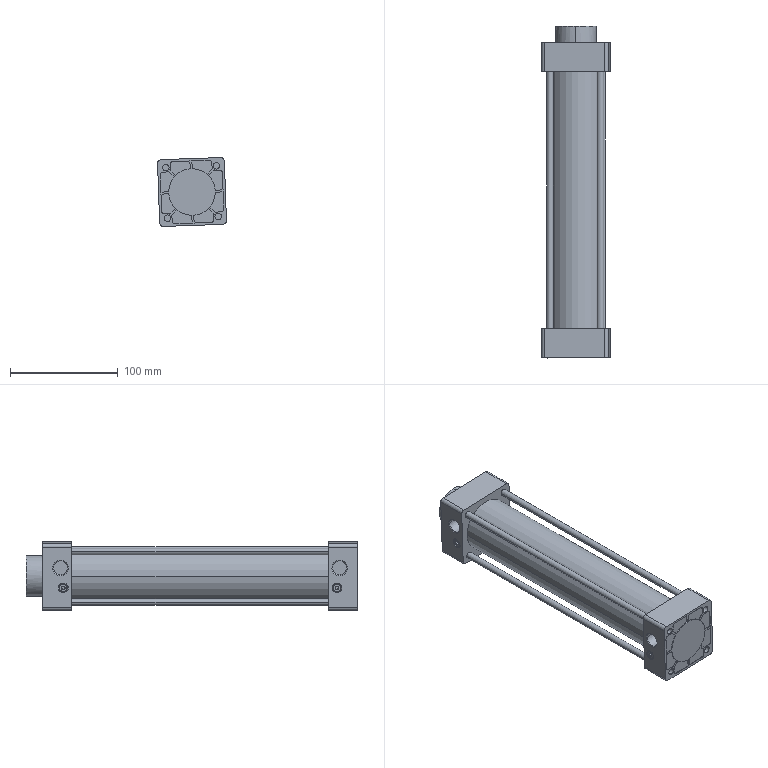Component | SolidWorks | ColumnLiftingCylinderSC50x200-1_ColumnLiftingCylinderBody-1 | 1 solid | 228 faces | box 63.91 x 308 x 63.91 mm | volume 626491 mm3 | plane 118 | cylinder 102 | cone 8 | commonest cylinder face diameters 6 x24 4.96 x16 43.32 x16 8.4 x16 6.2 x8 3.4 x4 6.8 x4 8 x4